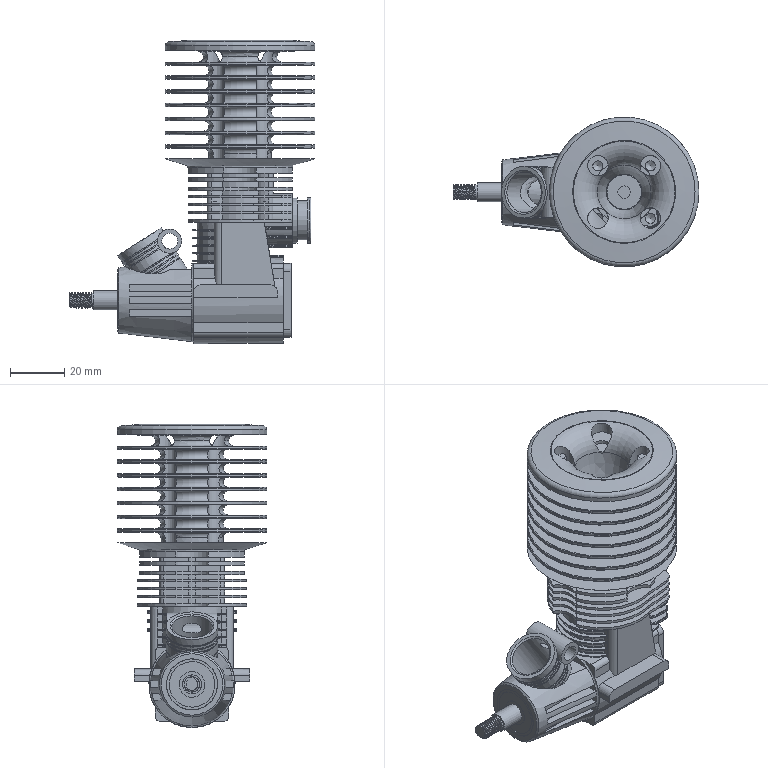Assembly | NX | mm | 11 component files | 17 solids | 795 faces | box 90.45 x 55.04 x 111.48 mm | volume 92358 mm3 | cylinder 349 | plane 313 | torus 86 | cone 24 | spline 23 | commonest cylinder face diameters 0.508 x34 2.794 x28 13.394 x28 24.292 x24 13.97 x22 5.08 x20 3.746 x12 40.132 x12
Bill of materials:
unnamed part 1 | 1 |  | Plain solid cylindrical rod with flat ends; looks like a straight pin or short round bar.
unnamed part 2 | 1 |  | Stepped shaft with a threaded small-diameter end, a plain journal, a larger hollow cylindrical section with a side window/port opening, and a counterweighted disc web at the other end carrying an offset small pin with a tiny axial hole. Looks like a crankshaft.
unnamed part 3 | 1 |  | Thin circular flange disc with a central boss projecting on both faces, a central through bore and four through holes on a bolt circle. Looks like a hub/drive flange.
unnamed part 4 | 1 |  | Cylindrical finned body: a stack of thin, evenly spaced circumferential fins around a core, with a thicker top plate whose top face is dished, a large central opening and four smaller holes. Looks like a finned cylinder head or heat sink.
unnamed part 5 | 1 |  | Hollow round tube with a square mounting flange at one end. The flange has rounded corners and four countersunk/chamfered corner holes, and there is a circumferential groove between tube and flange.
unnamed part 6 | 1 |  | Link with two ring-shaped ends (different sizes) joined by a slightly curved beam with a recessed/ribbed (I-section-like) web. Looks like a connecting rod.
unnamed part 7 | 1 |  | Thick plain annular ring with a central bore and flat faces. Faint concentric lines on the face suggest a separate inner and outer ring, like a simple ball-bearing representation.
unnamed part 8 | 1 |  | Solid cylindrical cup-like body with a flat closed top, a fine circumferential groove near the top, a transverse cross hole through the side walls, and a large notch cut from one side of the lower skirt. Looks like a piston.
unnamed part 9 | 1 |  | Thin-walled open tube with an outward flange/lip at the top end and rectangular port windows through the side wall at mid-height. Looks like a cylinder liner/sleeve.
unnamed part 10 | 1 |  | Flat annular disc/ring with a central hole relatively small compared to the outer diameter. Washer-like, or a ring like unnamed part 7 with a smaller bore.
unnamed part 11 | 1 |  | Complex housing: a finned vertical cylinder section with a top flange (four holes, large central bore), a lower crankcase body with a large rear circular opening and mounting holes, a forward tapered nose housing with a bore, side lugs, an angled tubular boss with an eyelet, and a short flanged side spigot. Looks like a small engine crankcase/cylinder casting.
Mates:
1. touch align | FinalBlock 1 face | BearingBig 1 face
2. touch align | BearingBig 1 face | FinalBlock 1 face
3. touch align | BearingSmall 1 face | FinalBlock 1 face
4. fix | FinalBlock 1 component
5. touch align | Sneider_CrankShaft 1 face | BearingSmall 1 face
6. touch align | Sneider_CrankShaft 1 face | BearingBig 1 face
7. touch align | BearingSmall 1 face | FinalBlock 1 face
8. touch align | Sneider_Sleeve 1 face | FinalBlock 1 face
9. touch align | Sneider_Sleeve 1 face | FinalBlock 1 face
10. touch align | Sneider_ConnectingRod 1 face | Sneider_CrankShaft 1 face
11. touch align | Sneider_ConnectingRod 1 face | Sneider_CrankShaft 1 face
12. touch align | Sneider_Piston 1 face | Sneider_Sleeve 1 face
13. touch align | Sneider_Piston 1 face | Sneider_ConnectingRod 1 face
14. touch align | Sneider_Pistonpin1 1 face | Sneider_ConnectingRod 1 face
15. center | Sneider_Pistonpin1 1 face | Sneider_Pistonpin1 1 face | Sneider_Piston 1 face
16. touch align | Sneider_backplate4Hole 1 face | FinalBlock 1 face
17. concentric | Sneider_backplate4Hole 1 edge | FinalBlock 1 edge
18. touch align | FinalBlock 1 face | Sneider_backplate4Hole 1 edge
19. touch align | Sneider__Head 1 face | FinalBlock 1 face
20. touch align | Sneider__Head 1 face | FinalBlock 1 edge
21. touch align | Sneider__Head 1 face | FinalBlock 1 face
22. touch align | Sneider__heat_sink 1 face | Sneider__Head 1 face
23. touch align | Sneider__heat_sink 1 edge | Sneider__Head 1 face
24. touch align | Sneider__heat_sink 1 face | Sneider__Head 1 face